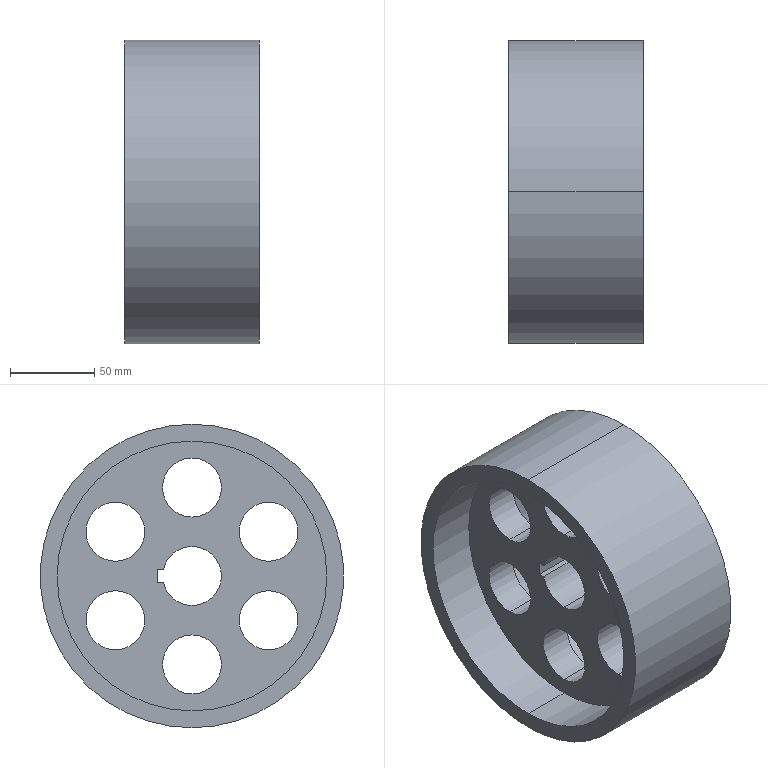Component | SolidWorks | ElectricalBoxAssembly2-1_GuideWheel-1 | 1 solid | 31 faces | box 80 x 180 x 180 mm | volume 723399 mm3 | cylinder 23 | plane 8 | commonest cylinder face diameters 35 x15 160 x4 50 x2 180 x2
STEP:
#1=COLOUR_RGB('',0.7922,0.8196,0.9333);
#2=FILL_AREA_STYLE_COLOUR('',#1);
#3=FILL_AREA_STYLE('',(#2));
#4=SURFACE_STYLE_FILL_AREA(#3);
#5=SURFACE_SIDE_STYLE('',(#4));
#6=SURFACE_STYLE_USAGE(.BOTH.,#5);
#7=PRESENTATION_STYLE_ASSIGNMENT((#6));
#8=CARTESIAN_POINT('',(28.68,8.451,56.945));
#9=VERTEX_POINT('',#8);
#10=CARTESIAN_POINT('',(28.68,8.451,63.244));
#11=VERTEX_POINT('',#10);
#12=CARTESIAN_POINT('',(28.68,8.451,60.094));
#13=DIRECTION('',(1.,0.,0.));
#14=DIRECTION('',(0.,0.,1.));
#15=AXIS2_PLACEMENT_3D('',#12,#13,#14);
#16=CIRCLE('',#15,3.15);
#17=EDGE_CURVE('',#9,#11,#16,.T.);
#18=ORIENTED_EDGE('',*,*,#17,.T.);
#19=CARTESIAN_POINT('',(27.499,8.451,63.244));
#20=VERTEX_POINT('',#19);
#21=CARTESIAN_POINT('',(28.68,8.451,63.244));
#22=DIRECTION('',(-1.,-0.,-0.));
#23=VECTOR('',#22,39.37);
#24=LINE('',#21,#23);
#25=EDGE_CURVE('',#11,#20,#24,.T.);
#26=ORIENTED_EDGE('',*,*,#25,.T.);
#27=CARTESIAN_POINT('',(27.499,8.451,56.945));
#28=VERTEX_POINT('',#27);
#29=CARTESIAN_POINT('',(27.499,8.451,60.094));
#30=DIRECTION('',(1.,0.,0.));
#31=DIRECTION('',(0.,0.,1.));
#32=AXIS2_PLACEMENT_3D('',#29,#30,#31);
#33=CIRCLE('',#32,3.15);
#34=EDGE_CURVE('',#28,#20,#33,.T.);
#35=ORIENTED_EDGE('',*,*,#34,.F.);
#36=CARTESIAN_POINT('',(28.68,8.451,56.945));
#37=DIRECTION('',(-1.,-0.,-0.));
#38=VECTOR('',#37,39.37);
#39=LINE('',#36,#38);
#40=EDGE_CURVE('',#9,#28,#39,.T.);
#41=ORIENTED_EDGE('',*,*,#40,.F.);
#42=EDGE_LOOP('',(#18,#26,#35,#41));
#43=FACE_OUTER_BOUND('',#42,.T.);
#44=CARTESIAN_POINT('',(28.68,8.451,60.094));
#45=DIRECTION('',(-1.,-0.,-0.));
#46=DIRECTION('',(0.,0.,-1.));
#47=AXIS2_PLACEMENT_3D('',#44,#45,#46);
#48=CYLINDRICAL_SURFACE('',#47,3.15);
#49=ADVANCED_FACE('',(#43),#48,.F.);
#50=CARTESIAN_POINT('',(27.499,10.241,61.817));
#51=VERTEX_POINT('',#50);
#52=CARTESIAN_POINT('',(27.499,10.241,60.439));
#53=VERTEX_POINT('',#52);
#54=CARTESIAN_POINT('',(27.499,10.241,61.128));
#55=DIRECTION('',(-1.,-0.,-0.));
#56=DIRECTION('',(0.,0.,-1.));
#57=AXIS2_PLACEMENT_3D('',#54,#55,#56);
#58=CIRCLE('',#57,0.689);
#59=EDGE_CURVE('',#51,#53,#58,.T.);
#60=ORIENTED_EDGE('',*,*,#59,.F.);
#61=CARTESIAN_POINT('',(26.711,10.241,61.817));
#62=VERTEX_POINT('',#61);
#63=CARTESIAN_POINT('',(28.68,10.241,61.817));
#64=DIRECTION('',(-1.,-0.,-0.));
#65=VECTOR('',#64,39.37);
#66=LINE('',#63,#65);
#67=EDGE_CURVE('',#51,#62,#66,.T.);
#68=ORIENTED_EDGE('',*,*,#67,.T.);
#69=CARTESIAN_POINT('',(26.711,10.241,60.439));
#70=VERTEX_POINT('',#69);
#71=CARTESIAN_POINT('',(26.711,10.241,61.128));
#72=DIRECTION('',(-1.,-0.,-0.));
#73=DIRECTION('',(0.,0.,-1.));
#74=AXIS2_PLACEMENT_3D('',#71,#72,#73);
#75=CIRCLE('',#74,0.689);
#76=EDGE_CURVE('',#62,#70,#75,.T.);
#77=ORIENTED_EDGE('',*,*,#76,.T.);
#78=CARTESIAN_POINT('',(28.68,10.241,60.439));
#79=DIRECTION('',(-1.,-0.,-0.));
#80=VECTOR('',#79,39.37);
#81=LINE('',#78,#80);
#82=EDGE_CURVE('',#53,#70,#81,.T.);
#83=ORIENTED_EDGE('',*,*,#82,.F.);
#84=EDGE_LOOP('',(#60,#68,#77,#83));
#85=FACE_OUTER_BOUND('',#84,.T.);
#86=CARTESIAN_POINT('',(28.68,10.241,61.128));
#87=DIRECTION('',(-1.,-0.,-0.));
#88=DIRECTION('',(0.,0.,-1.));
#89=AXIS2_PLACEMENT_3D('',#86,#87,#88);
#90=CYLINDRICAL_SURFACE('',#89,0.689);
#91=ADVANCED_FACE('',(#85),#90,.F.);
#92=CARTESIAN_POINT('',(27.499,10.241,59.75));
#93=VERTEX_POINT('',#92);
#94=CARTESIAN_POINT('',(27.499,10.241,58.372));
#95=VERTEX_POINT('',#94);
#96=CARTESIAN_POINT('',(27.499,10.241,59.061));
#97=DIRECTION('',(-1.,-0.,-0.));
#98=DIRECTION('',(0.,0.,-1.));
#99=AXIS2_PLACEMENT_3D('',#96,#97,#98);
#100=CIRCLE('',#99,0.689);
#101=EDGE_CURVE('',#93,#95,#100,.T.);
#102=ORIENTED_EDGE('',*,*,#101,.F.);
#103=CARTESIAN_POINT('',(26.711,10.241,59.75));
#104=VERTEX_POINT('',#103);
#105=CARTESIAN_POINT('',(28.68,10.241,59.75));
#106=DIRECTION('',(-1.,-0.,-0.));
#107=VECTOR('',#106,39.37);
#108=LINE('',#105,#107);
#109=EDGE_CURVE('',#93,#104,#108,.T.);
#110=ORIENTED_EDGE('',*,*,#109,.T.);
#111=CARTESIAN_POINT('',(26.711,10.241,58.372));
#112=VERTEX_POINT('',#111);
#113=CARTESIAN_POINT('',(26.711,10.241,59.061));
#114=DIRECTION('',(-1.,-0.,-0.));
#115=DIRECTION('',(0.,0.,-1.));
#116=AXIS2_PLACEMENT_3D('',#113,#114,#115);
#117=CIRCLE('',#116,0.689);
#118=EDGE_CURVE('',#104,#112,#117,.T.);
#119=ORIENTED_EDGE('',*,*,#118,.T.);
#120=CARTESIAN_POINT('',(28.68,10.241,58.372));
#121=DIRECTION('',(-1.,-0.,-0.));
#122=VECTOR('',#121,39.37);
#123=LINE('',#120,#122);
#124=EDGE_CURVE('',#95,#112,#123,.T.);
#125=ORIENTED_EDGE('',*,*,#124,.F.);
#126=EDGE_LOOP('',(#102,#110,#119,#125));
#127=FACE_OUTER_BOUND('',#126,.T.);
#128=CARTESIAN_POINT('',(28.68,10.241,59.061));
#129=DIRECTION('',(-1.,-0.,-0.));
#130=DIRECTION('',(0.,0.,-1.));
#131=AXIS2_PLACEMENT_3D('',#128,#129,#130);
#132=CYLINDRICAL_SURFACE('',#131,0.689);
#133=ADVANCED_FACE('',(#127),#132,.F.);
#134=CARTESIAN_POINT('',(27.499,8.451,58.716));
#135=VERTEX_POINT('',#134);
#136=CARTESIAN_POINT('',(27.499,8.451,57.339));
#137=VERTEX_POINT('',#136);
#138=CARTESIAN_POINT('',(27.499,8.451,58.028));
#139=DIRECTION('',(-1.,-0.,-0.));
#140=DIRECTION('',(0.,0.,-1.));
#141=AXIS2_PLACEMENT_3D('',#138,#139,#140);
#142=CIRCLE('',#141,0.689);
#143=EDGE_CURVE('',#135,#137,#142,.T.);
#144=ORIENTED_EDGE('',*,*,#143,.F.);
#145=CARTESIAN_POINT('',(26.711,8.451,58.716));
#146=VERTEX_POINT('',#145);
#147=CARTESIAN_POINT('',(28.68,8.451,58.716));
#148=DIRECTION('',(-1.,-0.,-0.));
#149=VECTOR('',#148,39.37);
#150=LINE('',#147,#149);
#151=EDGE_CURVE('',#135,#146,#150,.T.);
#152=ORIENTED_EDGE('',*,*,#151,.T.);
#153=CARTESIAN_POINT('',(26.711,8.451,57.339));
#154=VERTEX_POINT('',#153);
#155=CARTESIAN_POINT('',(26.711,8.451,58.028));
#156=DIRECTION('',(-1.,-0.,-0.));
#157=DIRECTION('',(0.,0.,-1.));
#158=AXIS2_PLACEMENT_3D('',#155,#156,#157);
#159=CIRCLE('',#158,0.689);
#160=EDGE_CURVE('',#146,#154,#159,.T.);
#161=ORIENTED_EDGE('',*,*,#160,.T.);
#162=CARTESIAN_POINT('',(28.68,8.451,57.339));
#163=DIRECTION('',(-1.,-0.,-0.));
#164=VECTOR('',#163,39.37);
#165=LINE('',#162,#164);
#166=EDGE_CURVE('',#137,#154,#165,.T.);
#167=ORIENTED_EDGE('',*,*,#166,.F.);
#168=EDGE_LOOP('',(#144,#152,#161,#167));
#169=FACE_OUTER_BOUND('',#168,.T.);
#170=CARTESIAN_POINT('',(28.68,8.451,58.028));
#171=DIRECTION('',(-1.,-0.,-0.));
#172=DIRECTION('',(0.,0.,-1.));
#173=AXIS2_PLACEMENT_3D('',#170,#171,#172);
#174=CYLINDRICAL_SURFACE('',#173,0.689);
#175=ADVANCED_FACE('',(#169),#174,.F.);
#176=CARTESIAN_POINT('',(27.499,6.661,59.75));
#177=VERTEX_POINT('',#176);
#178=CARTESIAN_POINT('',(27.499,6.661,58.372));
#179=VERTEX_POINT('',#178);
#180=CARTESIAN_POINT('',(27.499,6.661,59.061));
#181=DIRECTION('',(-1.,-0.,-0.));
#182=DIRECTION('',(0.,0.,-1.));
#183=AXIS2_PLACEMENT_3D('',#180,#181,#182);
#184=CIRCLE('',#183,0.689);
#185=EDGE_CURVE('',#177,#179,#184,.T.);
#186=ORIENTED_EDGE('',*,*,#185,.F.);
#187=CARTESIAN_POINT('',(26.711,6.661,59.75));
#188=VERTEX_POINT('',#187);
#189=CARTESIAN_POINT('',(28.68,6.661,59.75));
#190=DIRECTION('',(-1.,-0.,-0.));
#191=VECTOR('',#190,39.37);
#192=LINE('',#189,#191);
#193=EDGE_CURVE('',#177,#188,#192,.T.);
#194=ORIENTED_EDGE('',*,*,#193,.T.);
#195=CARTESIAN_POINT('',(26.711,6.661,58.372));
#196=VERTEX_POINT('',#195);
#197=CARTESIAN_POINT('',(26.711,6.661,59.061));
#198=DIRECTION('',(-1.,-0.,-0.));
#199=DIRECTION('',(0.,0.,-1.));
#200=AXIS2_PLACEMENT_3D('',#197,#198,#199);
#201=CIRCLE('',#200,0.689);
#202=EDGE_CURVE('',#188,#196,#201,.T.);
#203=ORIENTED_EDGE('',*,*,#202,.T.);
#204=CARTESIAN_POINT('',(28.68,6.661,58.372));
#205=DIRECTION('',(-1.,-0.,-0.));
#206=VECTOR('',#205,39.37);
#207=LINE('',#204,#206);
#208=EDGE_CURVE('',#179,#196,#207,.T.);
#209=ORIENTED_EDGE('',*,*,#208,.F.);
#210=EDGE_LOOP('',(#186,#194,#203,#209));
#211=FACE_OUTER_BOUND('',#210,.T.);
#212=CARTESIAN_POINT('',(28.68,6.661,59.061));
#213=DIRECTION('',(-1.,-0.,-0.));
#214=DIRECTION('',(0.,0.,-1.));
#215=AXIS2_PLACEMENT_3D('',#212,#213,#214);
#216=CYLINDRICAL_SURFACE('',#215,0.689);
#217=ADVANCED_FACE('',(#211),#216,.F.);
#218=CARTESIAN_POINT('',(27.499,6.661,61.817));
#219=VERTEX_POINT('',#218);
#220=CARTESIAN_POINT('',(27.499,6.661,60.439));
#221=VERTEX_POINT('',#220);
#222=CARTESIAN_POINT('',(27.499,6.661,61.128));
#223=DIRECTION('',(-1.,-0.,-0.));
#224=DIRECTION('',(0.,0.,-1.));
#225=AXIS2_PLACEMENT_3D('',#222,#223,#224);
#226=CIRCLE('',#225,0.689);
#227=EDGE_CURVE('',#219,#221,#226,.T.);
#228=ORIENTED_EDGE('',*,*,#227,.F.);
#229=CARTESIAN_POINT('',(26.711,6.661,61.817));
#230=VERTEX_POINT('',#229);
#231=CARTESIAN_POINT('',(28.68,6.661,61.817));
#232=DIRECTION('',(-1.,-0.,-0.));
#233=VECTOR('',#232,39.37);
#234=LINE('',#231,#233);
#235=EDGE_CURVE('',#219,#230,#234,.T.);
#236=ORIENTED_EDGE('',*,*,#235,.T.);
#237=CARTESIAN_POINT('',(26.711,6.661,60.439));
#238=VERTEX_POINT('',#237);
#239=CARTESIAN_POINT('',(26.711,6.661,61.128));
#240=DIRECTION('',(-1.,-0.,-0.));
#241=DIRECTION('',(0.,0.,-1.));
#242=AXIS2_PLACEMENT_3D('',#239,#240,#241);
#243=CIRCLE('',#242,0.689);
#244=EDGE_CURVE('',#230,#238,#243,.T.);
#245=ORIENTED_EDGE('',*,*,#244,.T.);
#246=CARTESIAN_POINT('',(28.68,6.661,60.439));
#247=DIRECTION('',(-1.,-0.,-0.));
#248=VECTOR('',#247,39.37);
#249=LINE('',#246,#248);
#250=EDGE_CURVE('',#221,#238,#249,.T.);
#251=ORIENTED_EDGE('',*,*,#250,.F.);
#252=EDGE_LOOP('',(#228,#236,#245,#251));
#253=FACE_OUTER_BOUND('',#252,.T.);
#254=CARTESIAN_POINT('',(28.68,6.661,61.128));
#255=DIRECTION('',(-1.,-0.,-0.));
#256=DIRECTION('',(0.,0.,-1.));
#257=AXIS2_PLACEMENT_3D('',#254,#255,#256);
#258=CYLINDRICAL_SURFACE('',#257,0.689);
#259=ADVANCED_FACE('',(#253),#258,.F.);
#260=CARTESIAN_POINT('',(27.499,8.451,62.85));
#261=VERTEX_POINT('',#260);
#262=CARTESIAN_POINT('',(27.499,8.451,61.472));
#263=VERTEX_POINT('',#262);
#264=CARTESIAN_POINT('',(27.499,8.451,62.161));
#265=DIRECTION('',(-1.,-0.,-0.));
#266=DIRECTION('',(0.,0.,-1.));
#267=AXIS2_PLACEMENT_3D('',#264,#265,#266);
#268=CIRCLE('',#267,0.689);
#269=EDGE_CURVE('',#261,#263,#268,.T.);
#270=ORIENTED_EDGE('',*,*,#269,.F.);
#271=CARTESIAN_POINT('',(26.711,8.451,62.85));
#272=VERTEX_POINT('',#271);
#273=CARTESIAN_POINT('',(28.68,8.451,62.85));
#274=DIRECTION('',(-1.,-0.,-0.));
#275=VECTOR('',#274,39.37);
#276=LINE('',#273,#275);
#277=EDGE_CURVE('',#261,#272,#276,.T.);
#278=ORIENTED_EDGE('',*,*,#277,.T.);
#279=CARTESIAN_POINT('',(26.711,8.451,61.472));
#280=VERTEX_POINT('',#279);
#281=CARTESIAN_POINT('',(26.711,8.451,62.161));
#282=DIRECTION('',(-1.,-0.,-0.));
#283=DIRECTION('',(0.,0.,-1.));
#284=AXIS2_PLACEMENT_3D('',#281,#282,#283);
#285=CIRCLE('',#284,0.689);
#286=EDGE_CURVE('',#272,#280,#285,.T.);
#287=ORIENTED_EDGE('',*,*,#286,.T.);
#288=CARTESIAN_POINT('',(28.68,8.451,61.472));
#289=DIRECTION('',(-1.,-0.,-0.));
#290=VECTOR('',#289,39.37);
#291=LINE('',#288,#290);
#292=EDGE_CURVE('',#263,#280,#291,.T.);
#293=ORIENTED_EDGE('',*,*,#292,.F.);
#294=EDGE_LOOP('',(#270,#278,#287,#293));
#295=FACE_OUTER_BOUND('',#294,.T.);
#296=CARTESIAN_POINT('',(28.68,8.451,62.161));
#297=DIRECTION('',(-1.,-0.,-0.));
#298=DIRECTION('',(0.,0.,-1.));
#299=AXIS2_PLACEMENT_3D('',#296,#297,#298);
#300=CYLINDRICAL_SURFACE('',#299,0.689);
#301=ADVANCED_FACE('',(#295),#300,.F.);
#302=CARTESIAN_POINT('',(26.711,8.451,63.244));
#303=VERTEX_POINT('',#302);
#304=CARTESIAN_POINT('',(26.711,8.451,56.945));
#305=VERTEX_POINT('',#304);
#306=CARTESIAN_POINT('',(26.711,8.451,60.094));
#307=DIRECTION('',(-1.,-0.,-0.));
#308=DIRECTION('',(0.,0.,-1.));
#309=AXIS2_PLACEMENT_3D('',#306,#307,#308);
#310=CIRCLE('',#309,3.15);
#311=EDGE_CURVE('',#303,#305,#310,.T.);
#312=ORIENTED_EDGE('',*,*,#311,.F.);
#313=CARTESIAN_POINT('',(25.53,8.451,63.244));
#314=VERTEX_POINT('',#313);
#315=CARTESIAN_POINT('',(26.711,8.451,63.244));
#316=DIRECTION('',(-1.,-0.,-0.));
#317=VECTOR('',#316,39.37);
#318=LINE('',#315,#317);
#319=EDGE_CURVE('',#303,#314,#318,.T.);
#320=ORIENTED_EDGE('',*,*,#319,.T.);
#321=CARTESIAN_POINT('',(25.53,8.451,56.945));
#322=VERTEX_POINT('',#321);
#323=CARTESIAN_POINT('',(25.53,8.451,60.094));
#324=DIRECTION('',(-1.,-0.,-0.));
#325=DIRECTION('',(0.,0.,-1.));
#326=AXIS2_PLACEMENT_3D('',#323,#324,#325);
#327=CIRCLE('',#326,3.15);
#328=EDGE_CURVE('',#314,#322,#327,.T.);
#329=ORIENTED_EDGE('',*,*,#328,.T.);
#330=CARTESIAN_POINT('',(26.711,8.451,56.945));
#331=DIRECTION('',(-1.,-0.,-0.));
#332=VECTOR('',#331,39.37);
#333=LINE('',#330,#332);
#334=EDGE_CURVE('',#305,#322,#333,.T.);
#335=ORIENTED_EDGE('',*,*,#334,.F.);
#336=EDGE_LOOP('',(#312,#320,#329,#335));
#337=FACE_OUTER_BOUND('',#336,.T.);
#338=CARTESIAN_POINT('',(26.711,8.451,60.094));
#339=DIRECTION('',(-1.,-0.,-0.));
#340=DIRECTION('',(0.,0.,-1.));
#341=AXIS2_PLACEMENT_3D('',#338,#339,#340);
#342=CYLINDRICAL_SURFACE('',#341,3.15);
#343=ADVANCED_FACE('',(#337),#342,.F.);
#344=CARTESIAN_POINT('',(28.68,8.451,59.11));
#345=VERTEX_POINT('',#344);
#346=CARTESIAN_POINT('',(28.68,8.451,61.079));
#347=VERTEX_POINT('',#346);
#348=CARTESIAN_POINT('',(28.68,8.451,60.094));
#349=DIRECTION('',(-1.,-0.,-0.));
#350=DIRECTION('',(0.,0.,-1.));
#351=AXIS2_PLACEMENT_3D('',#348,#349,#350);
#352=CIRCLE('',#351,0.9843);
#353=EDGE_CURVE('',#345,#347,#352,.T.);
#354=ORIENTED_EDGE('',*,*,#353,.T.);
#355=CARTESIAN_POINT('',(27.499,8.451,61.079));
#356=VERTEX_POINT('',#355);
#357=CARTESIAN_POINT('',(28.68,8.451,61.079));
#358=DIRECTION('',(-1.,-0.,-0.));
#359=VECTOR('',#358,39.37);
#360=LINE('',#357,#359);
#361=EDGE_CURVE('',#347,#356,#360,.T.);
#362=ORIENTED_EDGE('',*,*,#361,.T.);
#363=CARTESIAN_POINT('',(27.499,8.451,59.11));
#364=VERTEX_POINT('',#363);
#365=CARTESIAN_POINT('',(27.499,8.451,60.094));
#366=DIRECTION('',(-1.,-0.,-0.));
#367=DIRECTION('',(0.,0.,-1.));
#368=AXIS2_PLACEMENT_3D('',#365,#366,#367);
#369=CIRCLE('',#368,0.9843);
#370=EDGE_CURVE('',#364,#356,#369,.T.);
#371=ORIENTED_EDGE('',*,*,#370,.F.);
#372=CARTESIAN_POINT('',(28.68,8.451,59.11));
#373=DIRECTION('',(-1.,-0.,-0.));
#374=VECTOR('',#373,39.37);
#375=LINE('',#372,#374);
#376=EDGE_CURVE('',#345,#364,#375,.T.);
#377=ORIENTED_EDGE('',*,*,#376,.F.);
#378=EDGE_LOOP('',(#354,#362,#371,#377));
#379=FACE_OUTER_BOUND('',#378,.T.);
#380=CARTESIAN_POINT('',(28.68,8.451,60.094));
#381=DIRECTION('',(-1.,-0.,-0.));
#382=DIRECTION('',(0.,0.,-1.));
#383=AXIS2_PLACEMENT_3D('',#380,#381,#382);
#384=CYLINDRICAL_SURFACE('',#383,0.9843);
#385=ADVANCED_FACE('',(#379),#384,.T.);
#386=CARTESIAN_POINT('',(25.53,8.451,56.551));
#387=VERTEX_POINT('',#386);
#388=CARTESIAN_POINT('',(25.53,8.451,63.638));
#389=VERTEX_POINT('',#388);
#390=CARTESIAN_POINT('',(25.53,8.451,60.094));
#391=DIRECTION('',(-1.,-0.,-0.));
#392=DIRECTION('',(0.,0.,-1.));
#393=AXIS2_PLACEMENT_3D('',#390,#391,#392);
#394=CIRCLE('',#393,3.543);
#395=EDGE_CURVE('',#387,#389,#394,.T.);
#396=ORIENTED_EDGE('',*,*,#395,.F.);
#397=CARTESIAN_POINT('',(28.68,8.451,56.551));
#398=VERTEX_POINT('',#397);
#399=CARTESIAN_POINT('',(25.53,8.451,56.551));
#400=DIRECTION('',(1.,0.,0.));
#401=VECTOR('',#400,39.37);
#402=LINE('',#399,#401);
#403=EDGE_CURVE('',#387,#398,#402,.T.);
#404=ORIENTED_EDGE('',*,*,#403,.T.);
#405=CARTESIAN_POINT('',(28.68,8.451,63.638));
#406=VERTEX_POINT('',#405);
#407=CARTESIAN_POINT('',(28.68,8.451,60.094));
#408=DIRECTION('',(1.,0.,0.));
#409=DIRECTION('',(0.,0.,1.));
#410=AXIS2_PLACEMENT_3D('',#407,#408,#409);
#411=CIRCLE('',#410,3.543);
#412=EDGE_CURVE('',#406,#398,#411,.T.);
#413=ORIENTED_EDGE('',*,*,#412,.F.);
#414=CARTESIAN_POINT('',(25.53,8.451,63.638));
#415=DIRECTION('',(1.,0.,0.));
#416=VECTOR('',#415,39.37);
#417=LINE('',#414,#416);
#418=EDGE_CURVE('',#389,#406,#417,.T.);
#419=ORIENTED_EDGE('',*,*,#418,.F.);
#420=EDGE_LOOP('',(#396,#404,#413,#419));
#421=FACE_OUTER_BOUND('',#420,.T.);
#422=CARTESIAN_POINT('',(25.53,8.451,60.094));
#423=DIRECTION('',(1.,0.,0.));
#424=DIRECTION('',(0.,0.,1.));
#425=AXIS2_PLACEMENT_3D('',#422,#423,#424);
#426=CYLINDRICAL_SURFACE('',#425,3.543);
#427=ADVANCED_FACE('',(#421),#426,.T.);
#428=CARTESIAN_POINT('',(26.711,9.122,59.937));
#429=VERTEX_POINT('',#428);
#430=CARTESIAN_POINT('',(26.711,8.451,59.405));
#431=VERTEX_POINT('',#430);
#432=CARTESIAN_POINT('',(26.711,8.451,60.094));
#433=DIRECTION('',(-1.,-0.,-0.));
#434=DIRECTION('',(0.,0.,-1.));
#435=AXIS2_PLACEMENT_3D('',#432,#433,#434);
#436=CIRCLE('',#435,0.689);
#437=EDGE_CURVE('',#429,#431,#436,.T.);
#438=ORIENTED_EDGE('',*,*,#437,.T.);
#439=CARTESIAN_POINT('',(28.68,8.451,59.405));
#440=VERTEX_POINT('',#439);
#441=CARTESIAN_POINT('',(25.53,8.451,59.405));
#442=DIRECTION('',(1.,0.,0.));
#443=VECTOR('',#442,39.37);
#444=LINE('',#441,#443);
#445=EDGE_CURVE('',#431,#440,#444,.T.);
#446=ORIENTED_EDGE('',*,*,#445,.T.);
#447=CARTESIAN_POINT('',(28.68,9.122,59.937));
#448=VERTEX_POINT('',#447);
#449=CARTESIAN_POINT('',(28.68,8.451,60.094));
#450=DIRECTION('',(-1.,-0.,-0.));
#451=DIRECTION('',(0.,0.,-1.));
#452=AXIS2_PLACEMENT_3D('',#449,#450,#451);
#453=CIRCLE('',#452,0.689);
#454=EDGE_CURVE('',#448,#440,#453,.T.);
#455=ORIENTED_EDGE('',*,*,#454,.F.);
#456=CARTESIAN_POINT('',(25.53,9.122,59.937));
#457=DIRECTION('',(1.,0.,0.));
#458=VECTOR('',#457,39.37);
#459=LINE('',#456,#458);
#460=EDGE_CURVE('',#429,#448,#459,.T.);
#461=ORIENTED_EDGE('',*,*,#460,.F.);
#462=EDGE_LOOP('',(#438,#446,#455,#461));
#463=FACE_OUTER_BOUND('',#462,.T.);
#464=CARTESIAN_POINT('',(25.53,8.451,60.094));
#465=DIRECTION('',(1.,0.,0.));
#466=DIRECTION('',(0.,0.,1.));
#467=AXIS2_PLACEMENT_3D('',#464,#465,#466);
#468=CYLINDRICAL_SURFACE('',#467,0.689);
#469=ADVANCED_FACE('',(#463),#468,.F.);
#470=ORIENTED_EDGE('',*,*,#445,.F.);
#471=CARTESIAN_POINT('',(26.711,8.451,60.783));
#472=VERTEX_POINT('',#471);
#473=CARTESIAN_POINT('',(26.711,8.451,60.094));
#474=DIRECTION('',(-1.,-0.,-0.));
#475=DIRECTION('',(0.,0.,-1.));
#476=AXIS2_PLACEMENT_3D('',#473,#474,#475);
#477=CIRCLE('',#476,0.689);
#478=EDGE_CURVE('',#431,#472,#477,.T.);
#479=ORIENTED_EDGE('',*,*,#478,.T.);
#480=CARTESIAN_POINT('',(28.68,8.451,60.783));
#481=VERTEX_POINT('',#480);
#482=CARTESIAN_POINT('',(25.53,8.451,60.783));
#483=DIRECTION('',(1.,0.,0.));
#484=VECTOR('',#483,39.37);
#485=LINE('',#482,#484);
#486=EDGE_CURVE('',#472,#481,#485,.T.);
#487=ORIENTED_EDGE('',*,*,#486,.T.);
#488=CARTESIAN_POINT('',(28.68,8.451,60.094));
#489=DIRECTION('',(-1.,-0.,-0.));
#490=DIRECTION('',(0.,0.,-1.));
#491=AXIS2_PLACEMENT_3D('',#488,#489,#490);
#492=CIRCLE('',#491,0.689);
#493=EDGE_CURVE('',#440,#481,#492,.T.);
#494=ORIENTED_EDGE('',*,*,#493,.F.);
#495=EDGE_LOOP('',(#470,#479,#487,#494));
#496=FACE_OUTER_BOUND('',#495,.T.);
#497=CARTESIAN_POINT('',(25.53,8.451,60.094));
#498=DIRECTION('',(1.,0.,0.));
#499=DIRECTION('',(0.,0.,1.));
#500=AXIS2_PLACEMENT_3D('',#497,#498,#499);
#501=CYLINDRICAL_SURFACE('',#500,0.689);
#502=ADVANCED_FACE('',(#496),#501,.F.);
#503=ORIENTED_EDGE('',*,*,#370,.T.);
#504=CARTESIAN_POINT('',(27.499,8.451,60.094));
#505=DIRECTION('',(-1.,-0.,-0.));
#506=DIRECTION('',(0.,0.,-1.));
#507=AXIS2_PLACEMENT_3D('',#504,#505,#506);
#508=CIRCLE('',#507,0.9843);
#509=EDGE_CURVE('',#356,#364,#508,.T.);
#510=ORIENTED_EDGE('',*,*,#509,.T.);
#511=EDGE_LOOP('',(#503,#510));
#512=FACE_BOUND('',#511,.T.);
#513=CARTESIAN_POINT('',(27.499,8.451,62.161));
#514=DIRECTION('',(-1.,-0.,-0.));
#515=DIRECTION('',(0.,0.,-1.));
#516=AXIS2_PLACEMENT_3D('',#513,#514,#515);
#517=CIRCLE('',#516,0.689);
#518=EDGE_CURVE('',#263,#261,#517,.T.);
#519=ORIENTED_EDGE('',*,*,#518,.T.);
#520=ORIENTED_EDGE('',*,*,#269,.T.);
#521=EDGE_LOOP('',(#519,#520));
#522=FACE_BOUND('',#521,.T.);
#523=CARTESIAN_POINT('',(27.499,6.661,61.128));
#524=DIRECTION('',(-1.,-0.,-0.));
#525=DIRECTION('',(0.,0.,-1.));
#526=AXIS2_PLACEMENT_3D('',#523,#524,#525);
#527=CIRCLE('',#526,0.689);
#528=EDGE_CURVE('',#221,#219,#527,.T.);
#529=ORIENTED_EDGE('',*,*,#528,.T.);
#530=ORIENTED_EDGE('',*,*,#227,.T.);
#531=EDGE_LOOP('',(#529,#530));
#532=FACE_BOUND('',#531,.T.);
#533=CARTESIAN_POINT('',(27.499,6.661,59.061));
#534=DIRECTION('',(-1.,-0.,-0.));
#535=DIRECTION('',(0.,0.,-1.));
#536=AXIS2_PLACEMENT_3D('',#533,#534,#535);
#537=CIRCLE('',#536,0.689);
#538=EDGE_CURVE('',#179,#177,#537,.T.);
#539=ORIENTED_EDGE('',*,*,#538,.T.);
#540=ORIENTED_EDGE('',*,*,#185,.T.);
#541=EDGE_LOOP('',(#539,#540));
#542=FACE_BOUND('',#541,.T.);
#543=CARTESIAN_POINT('',(27.499,8.451,58.028));
#544=DIRECTION('',(-1.,-0.,-0.));
#545=DIRECTION('',(0.,0.,-1.));
#546=AXIS2_PLACEMENT_3D('',#543,#544,#545);
#547=CIRCLE('',#546,0.689);
#548=EDGE_CURVE('',#137,#135,#547,.T.);
#549=ORIENTED_EDGE('',*,*,#548,.T.);
#550=ORIENTED_EDGE('',*,*,#143,.T.);
#551=EDGE_LOOP('',(#549,#550));
#552=FACE_BOUND('',#551,.T.);
#553=CARTESIAN_POINT('',(27.499,10.241,59.061));
#554=DIRECTION('',(-1.,-0.,-0.));
#555=DIRECTION('',(0.,0.,-1.));
#556=AXIS2_PLACEMENT_3D('',#553,#554,#555);
#557=CIRCLE('',#556,0.689);
#558=EDGE_CURVE('',#95,#93,#557,.T.);
#559=ORIENTED_EDGE('',*,*,#558,.T.);
#560=ORIENTED_EDGE('',*,*,#101,.T.);
#561=EDGE_LOOP('',(#559,#560));
#562=FACE_BOUND('',#561,.T.);
#563=CARTESIAN_POINT('',(27.499,10.241,61.128));
#564=DIRECTION('',(-1.,-0.,-0.));
#565=DIRECTION('',(0.,0.,-1.));
#566=AXIS2_PLACEMENT_3D('',#563,#564,#565);
#567=CIRCLE('',#566,0.689);
#568=EDGE_CURVE('',#53,#51,#567,.T.);
#569=ORIENTED_EDGE('',*,*,#568,.T.);
#570=ORIENTED_EDGE('',*,*,#59,.T.);
#571=EDGE_LOOP('',(#569,#570));
#572=FACE_BOUND('',#571,.T.);
#573=ORIENTED_EDGE('',*,*,#34,.T.);
#574=CARTESIAN_POINT('',(27.499,8.451,60.094));
#575=DIRECTION('',(1.,0.,0.));
#576=DIRECTION('',(0.,0.,1.));
#577=AXIS2_PLACEMENT_3D('',#574,#575,#576);
#578=CIRCLE('',#577,3.15);
#579=EDGE_CURVE('',#20,#28,#578,.T.);
#580=ORIENTED_EDGE('',*,*,#579,.T.);
#581=EDGE_LOOP('',(#573,#580));
#582=FACE_OUTER_BOUND('',#581,.T.);
#583=CARTESIAN_POINT('',(27.499,8.451,60.094));
#584=DIRECTION('',(-1.,-0.,-0.));
#585=DIRECTION('',(0.,-0.,-1.));
#586=AXIS2_PLACEMENT_3D('',#583,#584,#585);
#587=PLANE('',#586);
#588=ADVANCED_FACE('',(#512,#522,#532,#542,#552,#562,#572,#582),#587,.F.);
#589=ORIENTED_EDGE('',*,*,#486,.F.);
#590=CARTESIAN_POINT('',(26.711,9.122,60.252));
#591=VERTEX_POINT('',#590);
#592=CARTESIAN_POINT('',(26.711,8.451,60.094));
#593=DIRECTION('',(-1.,-0.,-0.));
#594=DIRECTION('',(0.,0.,-1.));
#595=AXIS2_PLACEMENT_3D('',#592,#593,#594);
#596=CIRCLE('',#595,0.689);
#597=EDGE_CURVE('',#472,#591,#596,.T.);
#598=ORIENTED_EDGE('',*,*,#597,.T.);
#599=CARTESIAN_POINT('',(28.68,9.122,60.252));
#600=VERTEX_POINT('',#599);
#601=CARTESIAN_POINT('',(25.53,9.122,60.252));
#602=DIRECTION('',(-1.,-0.,-0.));
#603=VECTOR('',#602,39.37);
#604=LINE('',#601,#603);
#605=EDGE_CURVE('',#600,#591,#604,.T.);
#606=ORIENTED_EDGE('',*,*,#605,.F.);
#607=CARTESIAN_POINT('',(28.68,8.451,60.094));
#608=DIRECTION('',(-1.,-0.,-0.));
#609=DIRECTION('',(0.,0.,-1.));
#610=AXIS2_PLACEMENT_3D('',#607,#608,#609);
#611=CIRCLE('',#610,0.689);
#612=EDGE_CURVE('',#481,#600,#611,.T.);
#613=ORIENTED_EDGE('',*,*,#612,.F.);
#614=EDGE_LOOP('',(#589,#598,#606,#613));
#615=FACE_OUTER_BOUND('',#614,.T.);
#616=CARTESIAN_POINT('',(25.53,8.451,60.094));
#617=DIRECTION('',(1.,0.,0.));
#618=DIRECTION('',(0.,0.,1.));
#619=AXIS2_PLACEMENT_3D('',#616,#617,#618);
#620=CYLINDRICAL_SURFACE('',#619,0.689);
#621=ADVANCED_FACE('',(#615),#620,.F.);
#622=CARTESIAN_POINT('',(28.68,9.265,60.252));
#623=VERTEX_POINT('',#622);
#624=CARTESIAN_POINT('',(28.68,9.265,59.937));
#625=VERTEX_POINT('',#624);
#626=CARTESIAN_POINT('',(28.68,9.265,60.252));
#627=DIRECTION('',(0.,-0.,-1.));
#628=VECTOR('',#627,39.37);
#629=LINE('',#626,#628);
#630=EDGE_CURVE('',#623,#625,#629,.T.);
#631=ORIENTED_EDGE('',*,*,#630,.T.);
#632=CARTESIAN_POINT('',(28.68,9.107,59.937));
#633=DIRECTION('',(-0.,-1.,0.));
#634=VECTOR('',#633,39.37);
#635=LINE('',#632,#634);
#636=EDGE_CURVE('',#625,#448,#635,.T.);
#637=ORIENTED_EDGE('',*,*,#636,.T.);
#638=ORIENTED_EDGE('',*,*,#454,.T.);
#639=ORIENTED_EDGE('',*,*,#493,.T.);
#640=ORIENTED_EDGE('',*,*,#612,.T.);
#641=CARTESIAN_POINT('',(28.68,9.265,60.252));
#642=DIRECTION('',(0.,1.,-0.));
#643=VECTOR('',#642,39.37);
#644=LINE('',#641,#643);
#645=EDGE_CURVE('',#600,#623,#644,.T.);
#646=ORIENTED_EDGE('',*,*,#645,.T.);
#647=EDGE_LOOP('',(#631,#637,#638,#639,#640,#646));
#648=FACE_BOUND('',#647,.T.);
#649=ORIENTED_EDGE('',*,*,#353,.F.);
#650=CARTESIAN_POINT('',(28.68,8.451,60.094));
#651=DIRECTION('',(-1.,-0.,-0.));
#652=DIRECTION('',(0.,0.,-1.));
#653=AXIS2_PLACEMENT_3D('',#650,#651,#652);
#654=CIRCLE('',#653,0.9843);
#655=EDGE_CURVE('',#347,#345,#654,.T.);
#656=ORIENTED_EDGE('',*,*,#655,.F.);
#657=EDGE_LOOP('',(#649,#656));
#658=FACE_OUTER_BOUND('',#657,.T.);
#659=CARTESIAN_POINT('',(28.68,8.451,60.094));
#660=DIRECTION('',(-1.,-0.,-0.));
#661=DIRECTION('',(0.,-0.,-1.));
#662=AXIS2_PLACEMENT_3D('',#659,#660,#661);
#663=PLANE('',#662);
#664=ADVANCED_FACE('',(#648,#658),#663,.F.);
#665=CARTESIAN_POINT('',(25.53,8.451,60.094));
#666=DIRECTION('',(-1.,-0.,-0.));
#667=DIRECTION('',(0.,0.,-1.));
#668=AXIS2_PLACEMENT_3D('',#665,#666,#667);
#669=CIRCLE('',#668,3.15);
#670=EDGE_CURVE('',#322,#314,#669,.T.);
#671=ORIENTED_EDGE('',*,*,#670,.F.);
#672=ORIENTED_EDGE('',*,*,#328,.F.);
#673=EDGE_LOOP('',(#671,#672));
#674=FACE_BOUND('',#673,.T.);
#675=CARTESIAN_POINT('',(25.53,8.451,60.094));
#676=DIRECTION('',(-1.,-0.,-0.));
#677=DIRECTION('',(0.,0.,-1.));
#678=AXIS2_PLACEMENT_3D('',#675,#676,#677);
#679=CIRCLE('',#678,3.543);
#680=EDGE_CURVE('',#389,#387,#679,.T.);
#681=ORIENTED_EDGE('',*,*,#680,.T.);
#682=ORIENTED_EDGE('',*,*,#395,.T.);
#683=EDGE_LOOP('',(#681,#682));
#684=FACE_OUTER_BOUND('',#683,.T.);
#685=CARTESIAN_POINT('',(25.53,8.451,60.094));
#686=DIRECTION('',(-1.,-0.,-0.));
#687=DIRECTION('',(0.,-0.,-1.));
#688=AXIS2_PLACEMENT_3D('',#685,#686,#687);
#689=PLANE('',#688);
#690=ADVANCED_FACE('',(#674,#684),#689,.T.);
#691=ORIENTED_EDGE('',*,*,#403,.F.);
#692=ORIENTED_EDGE('',*,*,#680,.F.);
#693=ORIENTED_EDGE('',*,*,#418,.T.);
#694=CARTESIAN_POINT('',(28.68,8.451,60.094));
#695=DIRECTION('',(1.,0.,0.));
#696=DIRECTION('',(0.,0.,1.));
#697=AXIS2_PLACEMENT_3D('',#694,#695,#696);
#698=CIRCLE('',#697,3.543);
#699=EDGE_CURVE('',#398,#406,#698,.T.);
#700=ORIENTED_EDGE('',*,*,#699,.F.);
#701=EDGE_LOOP('',(#691,#692,#693,#700));
#702=FACE_OUTER_BOUND('',#701,.T.);
#703=CARTESIAN_POINT('',(25.53,8.451,60.094));
#704=DIRECTION('',(1.,0.,0.));
#705=DIRECTION('',(0.,0.,1.));
#706=AXIS2_PLACEMENT_3D('',#703,#704,#705);
#707=CYLINDRICAL_SURFACE('',#706,3.543);
#708=ADVANCED_FACE('',(#702),#707,.T.);
#709=ORIENTED_EDGE('',*,*,#361,.F.);
#710=ORIENTED_EDGE('',*,*,#655,.T.);
#711=ORIENTED_EDGE('',*,*,#376,.T.);
#712=ORIENTED_EDGE('',*,*,#509,.F.);
#713=EDGE_LOOP('',(#709,#710,#711,#712));
#714=FACE_OUTER_BOUND('',#713,.T.);
#715=CARTESIAN_POINT('',(28.68,8.451,60.094));
#716=DIRECTION('',(-1.,-0.,-0.));
#717=DIRECTION('',(0.,0.,-1.));
#718=AXIS2_PLACEMENT_3D('',#715,#716,#717);
#719=CYLINDRICAL_SURFACE('',#718,0.9843);
#720=ADVANCED_FACE('',(#714),#719,.T.);
#721=ORIENTED_EDGE('',*,*,#319,.F.);
#722=CARTESIAN_POINT('',(26.711,8.451,60.094));
#723=DIRECTION('',(-1.,-0.,-0.));
#724=DIRECTION('',(0.,0.,-1.));
#725=AXIS2_PLACEMENT_3D('',#722,#723,#724);
#726=CIRCLE('',#725,3.15);
#727=EDGE_CURVE('',#305,#303,#726,.T.);
#728=ORIENTED_EDGE('',*,*,#727,.F.);
#729=ORIENTED_EDGE('',*,*,#334,.T.);
#730=ORIENTED_EDGE('',*,*,#670,.T.);
#731=EDGE_LOOP('',(#721,#728,#729,#730));
#732=FACE_OUTER_BOUND('',#731,.T.);
#733=CARTESIAN_POINT('',(26.711,8.451,60.094));
#734=DIRECTION('',(-1.,-0.,-0.));
#735=DIRECTION('',(0.,0.,-1.));
#736=AXIS2_PLACEMENT_3D('',#733,#734,#735);
#737=CYLINDRICAL_SURFACE('',#736,3.15);
#738=ADVANCED_FACE('',(#732),#737,.F.);
#739=CARTESIAN_POINT('',(26.711,10.241,61.128));
#740=DIRECTION('',(-1.,-0.,-0.));
#741=DIRECTION('',(0.,0.,-1.));
#742=AXIS2_PLACEMENT_3D('',#739,#740,#741);
#743=CIRCLE('',#742,0.689);
#744=EDGE_CURVE('',#70,#62,#743,.T.);
#745=ORIENTED_EDGE('',*,*,#744,.F.);
#746=ORIENTED_EDGE('',*,*,#76,.F.);
#747=EDGE_LOOP('',(#745,#746));
#748=FACE_BOUND('',#747,.T.);
#749=CARTESIAN_POINT('',(26.711,10.241,59.061));
#750=DIRECTION('',(-1.,-0.,-0.));
#751=DIRECTION('',(0.,0.,-1.));
#752=AXIS2_PLACEMENT_3D('',#749,#750,#751);
#753=CIRCLE('',#752,0.689);
#754=EDGE_CURVE('',#112,#104,#753,.T.);
#755=ORIENTED_EDGE('',*,*,#754,.F.);
#756=ORIENTED_EDGE('',*,*,#118,.F.);
#757=EDGE_LOOP('',(#755,#756));
#758=FACE_BOUND('',#757,.T.);
#759=CARTESIAN_POINT('',(26.711,8.451,58.028));
#760=DIRECTION('',(-1.,-0.,-0.));
#761=DIRECTION('',(0.,0.,-1.));
#762=AXIS2_PLACEMENT_3D('',#759,#760,#761);
#763=CIRCLE('',#762,0.689);
#764=EDGE_CURVE('',#154,#146,#763,.T.);
#765=ORIENTED_EDGE('',*,*,#764,.F.);
#766=ORIENTED_EDGE('',*,*,#160,.F.);
#767=EDGE_LOOP('',(#765,#766));
#768=FACE_BOUND('',#767,.T.);
#769=CARTESIAN_POINT('',(26.711,6.661,59.061));
#770=DIRECTION('',(-1.,-0.,-0.));
#771=DIRECTION('',(0.,0.,-1.));
#772=AXIS2_PLACEMENT_3D('',#769,#770,#771);
#773=CIRCLE('',#772,0.689);
#774=EDGE_CURVE('',#196,#188,#773,.T.);
#775=ORIENTED_EDGE('',*,*,#774,.F.);
#776=ORIENTED_EDGE('',*,*,#202,.F.);
#777=EDGE_LOOP('',(#775,#776));
#778=FACE_BOUND('',#777,.T.);
#779=CARTESIAN_POINT('',(26.711,6.661,61.128));
#780=DIRECTION('',(-1.,-0.,-0.));
#781=DIRECTION('',(0.,0.,-1.));
#782=AXIS2_PLACEMENT_3D('',#779,#780,#781);
#783=CIRCLE('',#782,0.689);
#784=EDGE_CURVE('',#238,#230,#783,.T.);
#785=ORIENTED_EDGE('',*,*,#784,.F.);
#786=ORIENTED_EDGE('',*,*,#244,.F.);
#787=EDGE_LOOP('',(#785,#786));
#788=FACE_BOUND('',#787,.T.);
#789=CARTESIAN_POINT('',(26.711,9.265,59.937));
#790=VERTEX_POINT('',#789);
#791=CARTESIAN_POINT('',(26.711,9.107,59.937));
#792=DIRECTION('',(-0.,-1.,0.));
#793=VECTOR('',#792,39.37);
#794=LINE('',#791,#793);
#795=EDGE_CURVE('',#790,#429,#794,.T.);
#796=ORIENTED_EDGE('',*,*,#795,.F.);
#797=CARTESIAN_POINT('',(26.711,9.265,60.252));
#798=VERTEX_POINT('',#797);
#799=CARTESIAN_POINT('',(26.711,9.265,60.252));
#800=DIRECTION('',(0.,-0.,-1.));
#801=VECTOR('',#800,39.37);
#802=LINE('',#799,#801);
#803=EDGE_CURVE('',#798,#790,#802,.T.);
#804=ORIENTED_EDGE('',*,*,#803,.F.);
#805=CARTESIAN_POINT('',(26.711,8.451,60.252));
#806=DIRECTION('',(0.,1.,-0.));
#807=VECTOR('',#806,39.37);
#808=LINE('',#805,#807);
#809=EDGE_CURVE('',#591,#798,#808,.T.);
#810=ORIENTED_EDGE('',*,*,#809,.F.);
#811=ORIENTED_EDGE('',*,*,#597,.F.);
#812=ORIENTED_EDGE('',*,*,#478,.F.);
#813=ORIENTED_EDGE('',*,*,#437,.F.);
#814=EDGE_LOOP('',(#796,#804,#810,#811,#812,#813));
#815=FACE_BOUND('',#814,.T.);
#816=CARTESIAN_POINT('',(26.711,8.451,62.161));
#817=DIRECTION('',(-1.,-0.,-0.));
#818=DIRECTION('',(0.,0.,-1.));
#819=AXIS2_PLACEMENT_3D('',#816,#817,#818);
#820=CIRCLE('',#819,0.689);
#821=EDGE_CURVE('',#280,#272,#820,.T.);
#822=ORIENTED_EDGE('',*,*,#821,.F.);
#823=ORIENTED_EDGE('',*,*,#286,.F.);
#824=EDGE_LOOP('',(#822,#823));
#825=FACE_BOUND('',#824,.T.);
#826=ORIENTED_EDGE('',*,*,#727,.T.);
#827=ORIENTED_EDGE('',*,*,#311,.T.);
#828=EDGE_LOOP('',(#826,#827));
#829=FACE_OUTER_BOUND('',#828,.T.);
#830=CARTESIAN_POINT('',(26.711,8.451,60.094));
#831=DIRECTION('',(-1.,-0.,-0.));
#832=DIRECTION('',(0.,-0.,-1.));
#833=AXIS2_PLACEMENT_3D('',#830,#831,#832);
#834=PLANE('',#833);
#835=ADVANCED_FACE('',(#748,#758,#768,#778,#788,#815,#825,#829),#834,.T.);
#836=ORIENTED_EDGE('',*,*,#277,.F.);
#837=ORIENTED_EDGE('',*,*,#518,.F.);
#838=ORIENTED_EDGE('',*,*,#292,.T.);
#839=ORIENTED_EDGE('',*,*,#821,.T.);
#840=EDGE_LOOP('',(#836,#837,#838,#839));
#841=FACE_OUTER_BOUND('',#840,.T.);
#842=CARTESIAN_POINT('',(28.68,8.451,62.161));
#843=DIRECTION('',(-1.,-0.,-0.));
#844=DIRECTION('',(0.,0.,-1.));
#845=AXIS2_PLACEMENT_3D('',#842,#843,#844);
#846=CYLINDRICAL_SURFACE('',#845,0.689);
#847=ADVANCED_FACE('',(#841),#846,.F.);
#848=ORIENTED_EDGE('',*,*,#460,.T.);
#849=ORIENTED_EDGE('',*,*,#636,.F.);
#850=CARTESIAN_POINT('',(28.68,9.265,59.937));
#851=DIRECTION('',(-1.,-0.,-0.));
#852=VECTOR('',#851,39.37);
#853=LINE('',#850,#852);
#854=EDGE_CURVE('',#625,#790,#853,.T.);
#855=ORIENTED_EDGE('',*,*,#854,.T.);
#856=ORIENTED_EDGE('',*,*,#795,.T.);
#857=EDGE_LOOP('',(#848,#849,#855,#856));
#858=FACE_OUTER_BOUND('',#857,.T.);
#859=CARTESIAN_POINT('',(28.68,9.107,59.937));
#860=DIRECTION('',(0.,-0.,-1.));
#861=DIRECTION('',(-0.,-1.,0.));
#862=AXIS2_PLACEMENT_3D('',#859,#860,#861);
#863=PLANE('',#862);
#864=ADVANCED_FACE('',(#858),#863,.F.);
#865=ORIENTED_EDGE('',*,*,#803,.T.);
#866=ORIENTED_EDGE('',*,*,#854,.F.);
#867=ORIENTED_EDGE('',*,*,#630,.F.);
#868=CARTESIAN_POINT('',(28.68,9.265,60.252));
#869=DIRECTION('',(-1.,-0.,-0.));
#870=VECTOR('',#869,39.37);
#871=LINE('',#868,#870);
#872=EDGE_CURVE('',#623,#798,#871,.T.);
#873=ORIENTED_EDGE('',*,*,#872,.T.);
#874=EDGE_LOOP('',(#865,#866,#867,#873));
#875=FACE_OUTER_BOUND('',#874,.T.);
#876=CARTESIAN_POINT('',(28.68,9.265,60.252));
#877=DIRECTION('',(-0.,1.,0.));
#878=DIRECTION('',(1.,0.,0.));
#879=AXIS2_PLACEMENT_3D('',#876,#877,#878);
#880=PLANE('',#879);
#881=ADVANCED_FACE('',(#875),#880,.F.);
#882=ORIENTED_EDGE('',*,*,#605,.T.);
#883=ORIENTED_EDGE('',*,*,#809,.T.);
#884=ORIENTED_EDGE('',*,*,#872,.F.);
#885=ORIENTED_EDGE('',*,*,#645,.F.);
#886=EDGE_LOOP('',(#882,#883,#884,#885));
#887=FACE_OUTER_BOUND('',#886,.T.);
#888=CARTESIAN_POINT('',(28.68,9.265,60.252));
#889=DIRECTION('',(-0.,0.,1.));
#890=DIRECTION('',(0.,1.,-0.));
#891=AXIS2_PLACEMENT_3D('',#888,#889,#890);
#892=PLANE('',#891);
#893=ADVANCED_FACE('',(#887),#892,.F.);
#894=ORIENTED_EDGE('',*,*,#235,.F.);
#895=ORIENTED_EDGE('',*,*,#528,.F.);
#896=ORIENTED_EDGE('',*,*,#250,.T.);
#897=ORIENTED_EDGE('',*,*,#784,.T.);
#898=EDGE_LOOP('',(#894,#895,#896,#897));
#899=FACE_OUTER_BOUND('',#898,.T.);
#900=CARTESIAN_POINT('',(28.68,6.661,61.128));
#901=DIRECTION('',(-1.,-0.,-0.));
#902=DIRECTION('',(0.,0.,-1.));
#903=AXIS2_PLACEMENT_3D('',#900,#901,#902);
#904=CYLINDRICAL_SURFACE('',#903,0.689);
#905=ADVANCED_FACE('',(#899),#904,.F.);
#906=ORIENTED_EDGE('',*,*,#193,.F.);
#907=ORIENTED_EDGE('',*,*,#538,.F.);
#908=ORIENTED_EDGE('',*,*,#208,.T.);
#909=ORIENTED_EDGE('',*,*,#774,.T.);
#910=EDGE_LOOP('',(#906,#907,#908,#909));
#911=FACE_OUTER_BOUND('',#910,.T.);
#912=CARTESIAN_POINT('',(28.68,6.661,59.061));
#913=DIRECTION('',(-1.,-0.,-0.));
#914=DIRECTION('',(0.,0.,-1.));
#915=AXIS2_PLACEMENT_3D('',#912,#913,#914);
#916=CYLINDRICAL_SURFACE('',#915,0.689);
#917=ADVANCED_FACE('',(#911),#916,.F.);
#918=ORIENTED_EDGE('',*,*,#151,.F.);
#919=ORIENTED_EDGE('',*,*,#548,.F.);
#920=ORIENTED_EDGE('',*,*,#166,.T.);
#921=ORIENTED_EDGE('',*,*,#764,.T.);
#922=EDGE_LOOP('',(#918,#919,#920,#921));
#923=FACE_OUTER_BOUND('',#922,.T.);
#924=CARTESIAN_POINT('',(28.68,8.451,58.028));
#925=DIRECTION('',(-1.,-0.,-0.));
#926=DIRECTION('',(0.,0.,-1.));
#927=AXIS2_PLACEMENT_3D('',#924,#925,#926);
#928=CYLINDRICAL_SURFACE('',#927,0.689);
#929=ADVANCED_FACE('',(#923),#928,.F.);
#930=ORIENTED_EDGE('',*,*,#109,.F.);
#931=ORIENTED_EDGE('',*,*,#558,.F.);
#932=ORIENTED_EDGE('',*,*,#124,.T.);
#933=ORIENTED_EDGE('',*,*,#754,.T.);
#934=EDGE_LOOP('',(#930,#931,#932,#933));
#935=FACE_OUTER_BOUND('',#934,.T.);
#936=CARTESIAN_POINT('',(28.68,10.241,59.061));
#937=DIRECTION('',(-1.,-0.,-0.));
#938=DIRECTION('',(0.,0.,-1.));
#939=AXIS2_PLACEMENT_3D('',#936,#937,#938);
#940=CYLINDRICAL_SURFACE('',#939,0.689);
#941=ADVANCED_FACE('',(#935),#940,.F.);
#942=ORIENTED_EDGE('',*,*,#67,.F.);
#943=ORIENTED_EDGE('',*,*,#568,.F.);
#944=ORIENTED_EDGE('',*,*,#82,.T.);
#945=ORIENTED_EDGE('',*,*,#744,.T.);
#946=EDGE_LOOP('',(#942,#943,#944,#945));
#947=FACE_OUTER_BOUND('',#946,.T.);
#948=CARTESIAN_POINT('',(28.68,10.241,61.128));
#949=DIRECTION('',(-1.,-0.,-0.));
#950=DIRECTION('',(0.,0.,-1.));
#951=AXIS2_PLACEMENT_3D('',#948,#949,#950);
#952=CYLINDRICAL_SURFACE('',#951,0.689);
#953=ADVANCED_FACE('',(#947),#952,.F.);
#954=ORIENTED_EDGE('',*,*,#412,.T.);
#955=ORIENTED_EDGE('',*,*,#699,.T.);
#956=EDGE_LOOP('',(#954,#955));
#957=FACE_OUTER_BOUND('',#956,.T.);
#958=ORIENTED_EDGE('',*,*,#17,.F.);
#959=CARTESIAN_POINT('',(28.68,8.451,60.094));
#960=DIRECTION('',(1.,0.,0.));
#961=DIRECTION('',(0.,0.,1.));
#962=AXIS2_PLACEMENT_3D('',#959,#960,#961);
#963=CIRCLE('',#962,3.15);
#964=EDGE_CURVE('',#11,#9,#963,.T.);
#965=ORIENTED_EDGE('',*,*,#964,.F.);
#966=EDGE_LOOP('',(#958,#965));
#967=FACE_BOUND('',#966,.T.);
#968=CARTESIAN_POINT('',(28.68,8.451,60.094));
#969=DIRECTION('',(1.,0.,0.));
#970=DIRECTION('',(-0.,0.,1.));
#971=AXIS2_PLACEMENT_3D('',#968,#969,#970);
#972=PLANE('',#971);
#973=ADVANCED_FACE('',(#957,#967),#972,.T.);
#974=ORIENTED_EDGE('',*,*,#25,.F.);
#975=ORIENTED_EDGE('',*,*,#964,.T.);
#976=ORIENTED_EDGE('',*,*,#40,.T.);
#977=ORIENTED_EDGE('',*,*,#579,.F.);
#978=EDGE_LOOP('',(#974,#975,#976,#977));
#979=FACE_OUTER_BOUND('',#978,.T.);
#980=CARTESIAN_POINT('',(28.68,8.451,60.094));
#981=DIRECTION('',(-1.,-0.,-0.));
#982=DIRECTION('',(0.,0.,-1.));
#983=AXIS2_PLACEMENT_3D('',#980,#981,#982);
#984=CYLINDRICAL_SURFACE('',#983,3.15);
#985=ADVANCED_FACE('',(#979),#984,.F.);
#986=CLOSED_SHELL('',(#49,#91,#133,#175,#217,#259,#301,#343,#385,#427,#469,#502,#588,#621,#664,#690,#708,#720,#738,#835,#847,#864,#881,#893,#905,#917,#929,#941,#953,#973,#985));
#987=MANIFOLD_SOLID_BREP('',#986);
#988=STYLED_ITEM('',(#7),#987);
#989=(LENGTH_UNIT()NAMED_UNIT(*)SI_UNIT($,.METRE.));
#990=LENGTH_MEASURE_WITH_UNIT(LENGTH_MEASURE(0.0254),#989);
#991=DIMENSIONAL_EXPONENTS(1.,0.,0.,0.,0.,0.,0.);
#992=(CONVERSION_BASED_UNIT('',#990)LENGTH_UNIT()NAMED_UNIT(#991));
#993=UNCERTAINTY_MEASURE_WITH_UNIT(LENGTH_MEASURE(0.00001),#992,'','');
#994=(NAMED_UNIT(*)PLANE_ANGLE_UNIT()SI_UNIT($,.RADIAN.));
#995=(NAMED_UNIT(*)SI_UNIT($,.STERADIAN.)SOLID_ANGLE_UNIT());
#996=(GEOMETRIC_REPRESENTATION_CONTEXT(3)GLOBAL_UNCERTAINTY_ASSIGNED_CONTEXT((#993))GLOBAL_UNIT_ASSIGNED_CONTEXT((#992,#994,#995))REPRESENTATION_CONTEXT('',''));
#997=MECHANICAL_DESIGN_GEOMETRIC_PRESENTATION_REPRESENTATION('',(#988),#996);
#998=PRESENTATION_LAYER_ASSIGNMENT('','',(#988));
#999=CARTESIAN_POINT('',(0.,0.,0.));
#1000=DIRECTION('',(0.,0.,1.));
#1001=DIRECTION('',(1.,0.,0.));
#1002=AXIS2_PLACEMENT_3D('',#999,#1000,#1001);
#1003=(LENGTH_UNIT()NAMED_UNIT(*)SI_UNIT($,.METRE.));
#1004=LENGTH_MEASURE_WITH_UNIT(LENGTH_MEASURE(0.0254),#1003);
#1005=DIMENSIONAL_EXPONENTS(1.,0.,0.,0.,0.,0.,0.);
#1006=(CONVERSION_BASED_UNIT('',#1004)LENGTH_UNIT()NAMED_UNIT(#1005));
#1007=UNCERTAINTY_MEASURE_WITH_UNIT(LENGTH_MEASURE(0.00001),#1006,'','');
#1008=(NAMED_UNIT(*)PLANE_ANGLE_UNIT()SI_UNIT($,.RADIAN.));
#1009=(NAMED_UNIT(*)SI_UNIT($,.STERADIAN.)SOLID_ANGLE_UNIT());
#1010=(GEOMETRIC_REPRESENTATION_CONTEXT(3)GLOBAL_UNCERTAINTY_ASSIGNED_CONTEXT((#1007))GLOBAL_UNIT_ASSIGNED_CONTEXT((#1006,#1008,#1009))REPRESENTATION_CONTEXT('',''));
#1011=ADVANCED_BREP_SHAPE_REPRESENTATION('',(#987,#1002),#1010);